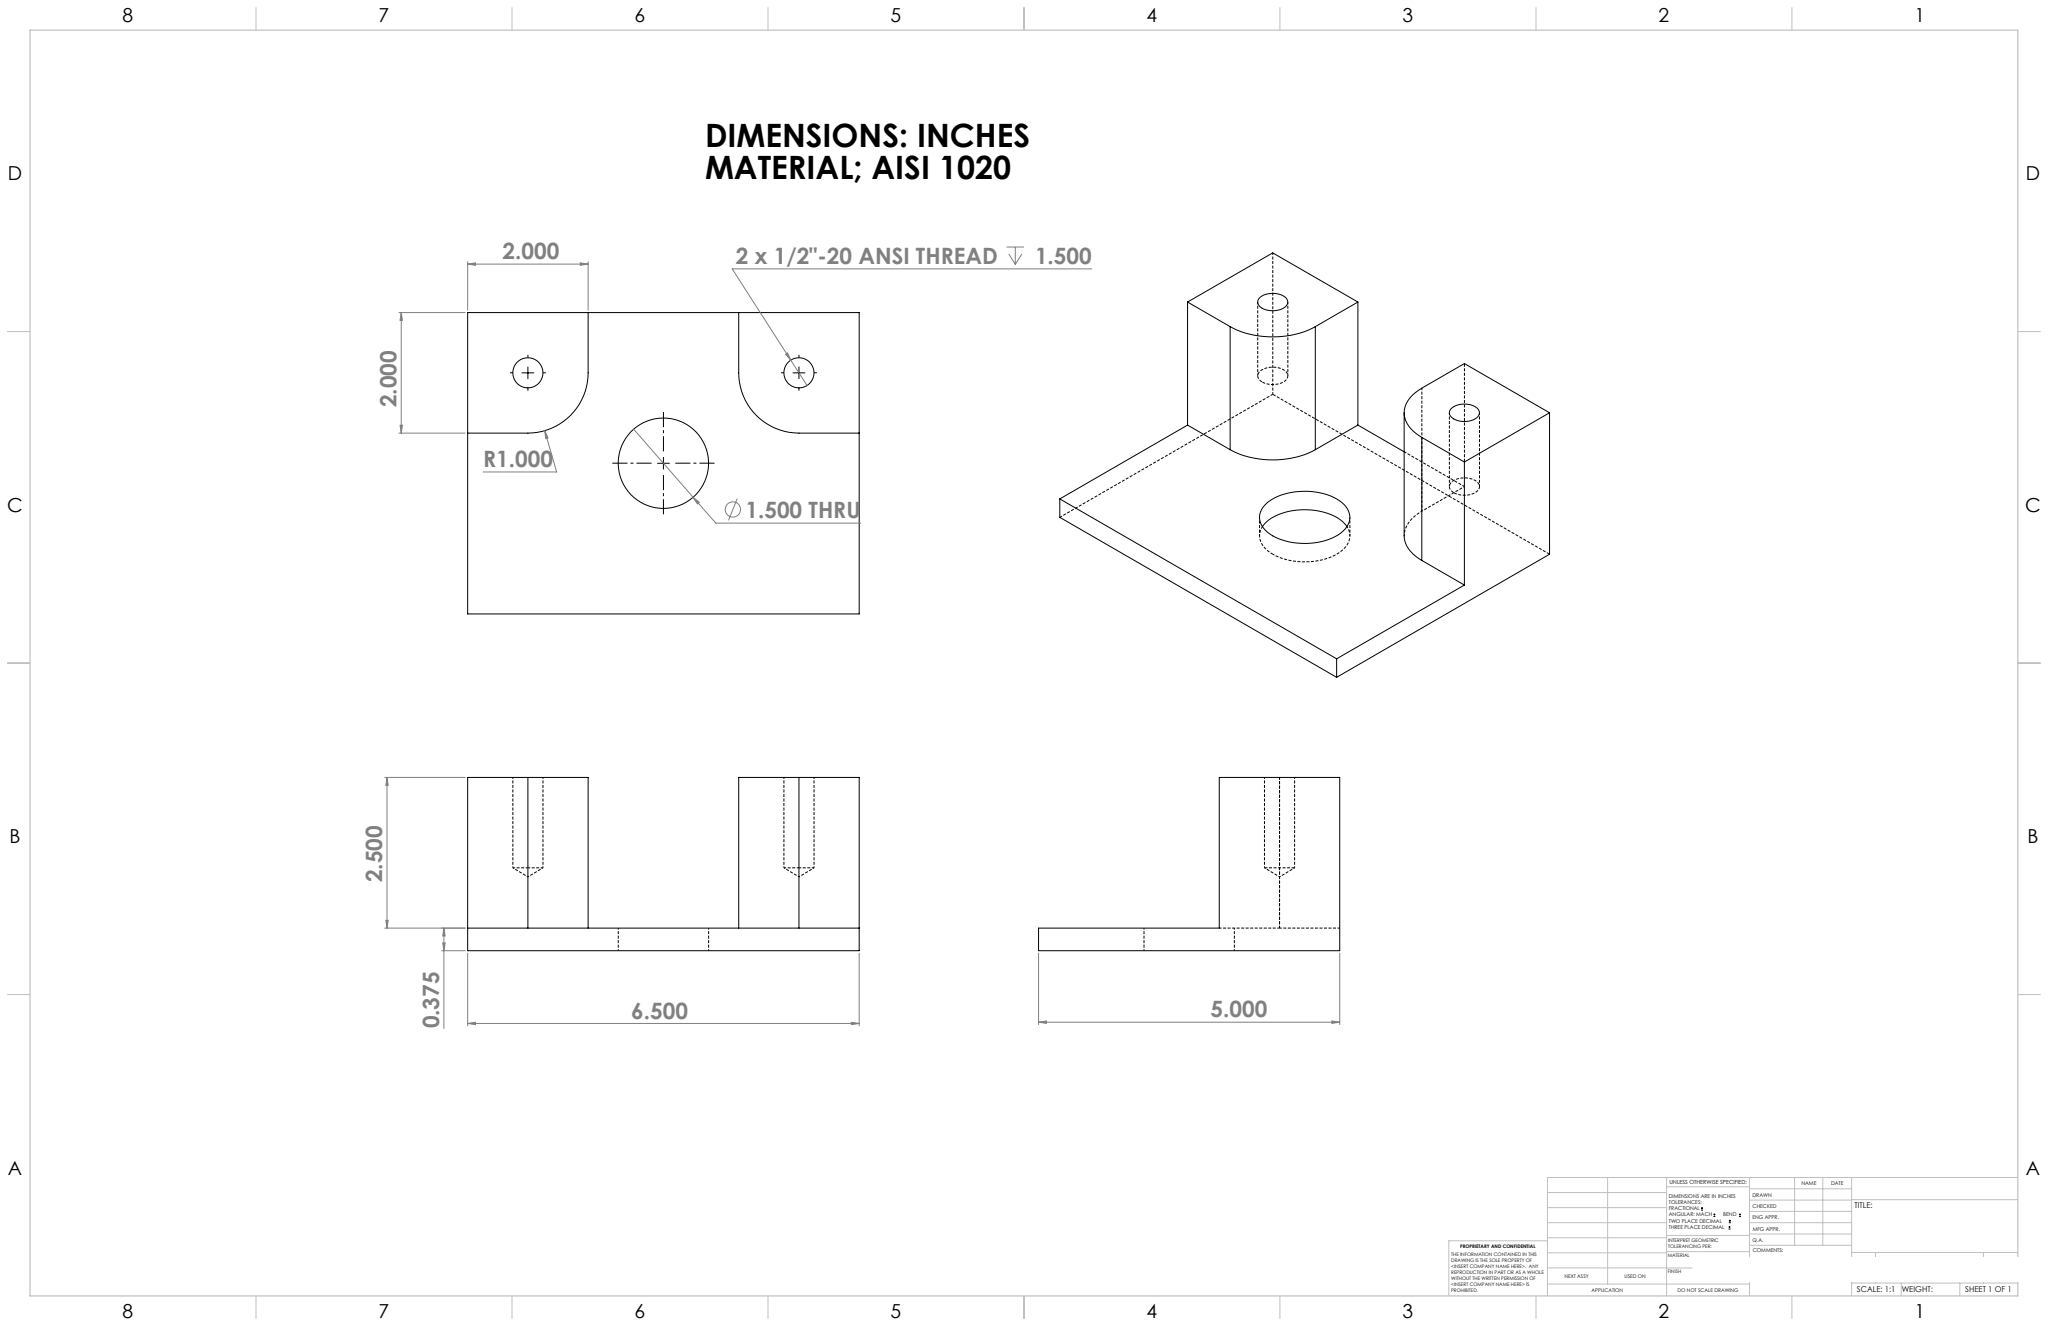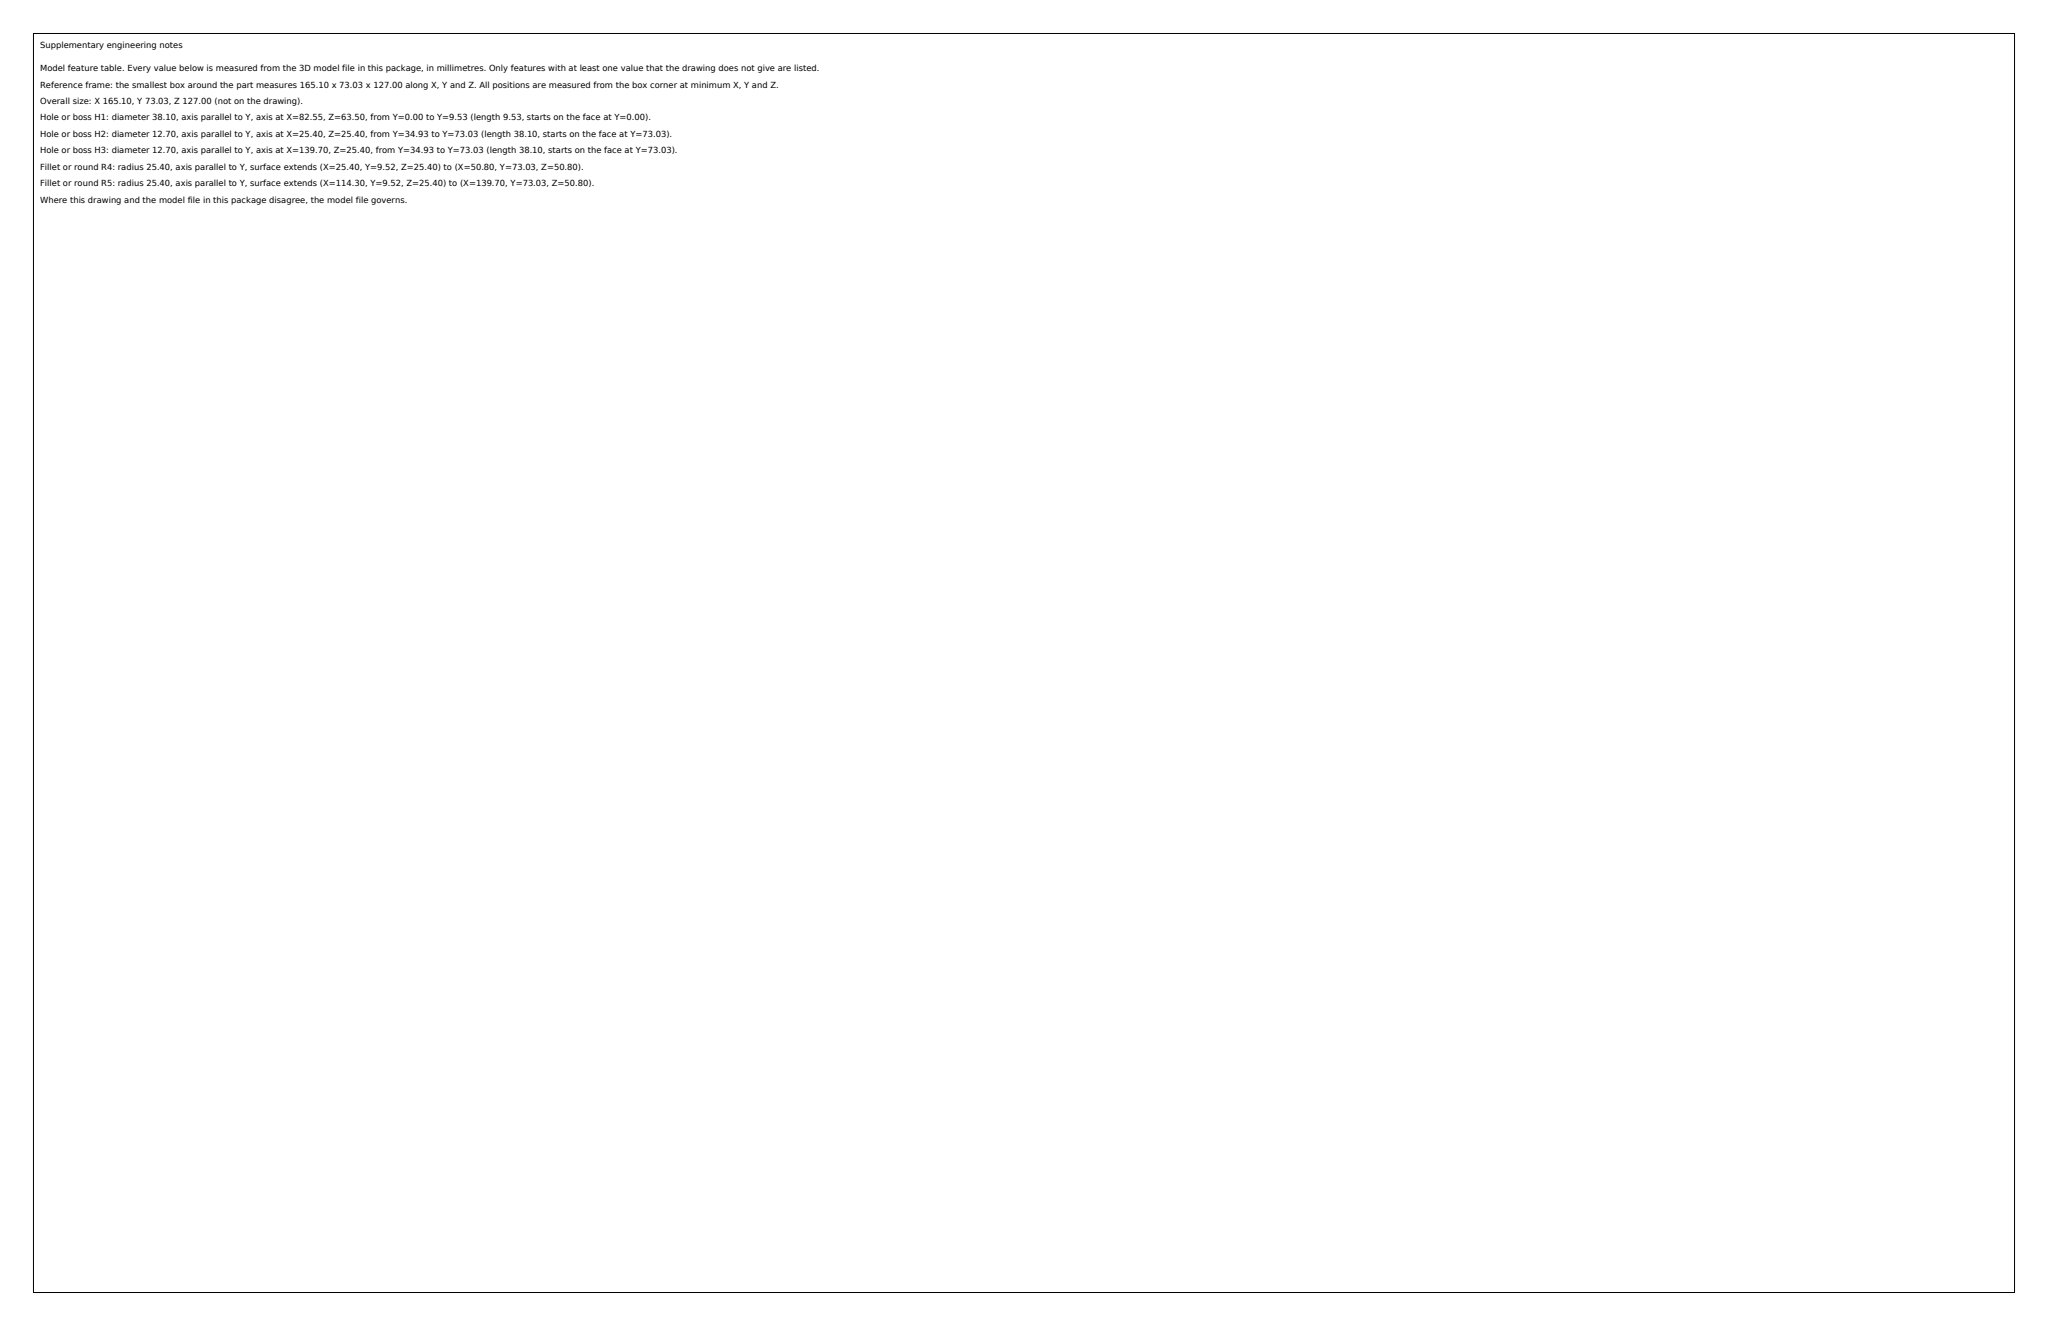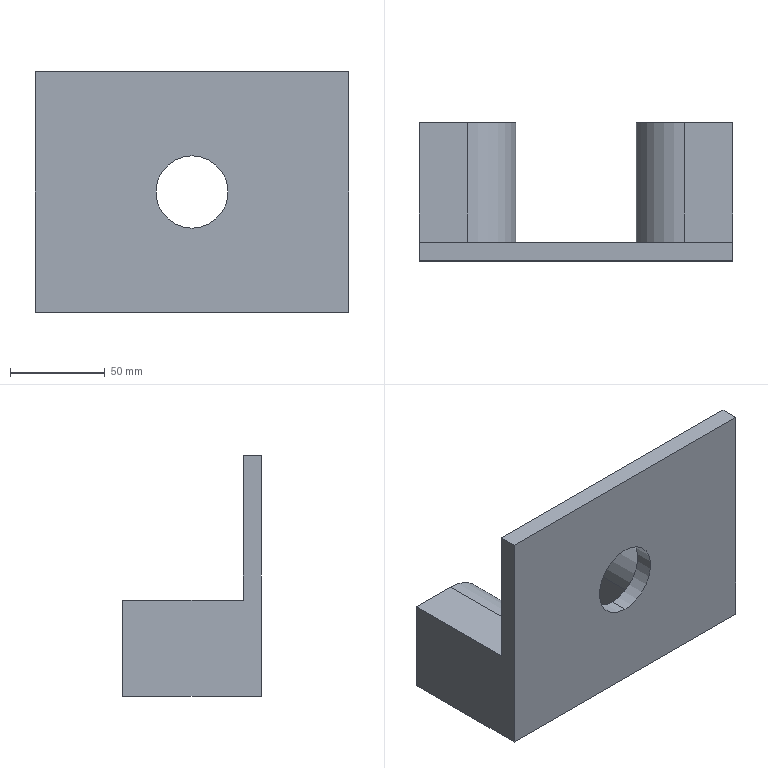Part | SolidWorks | mm | material AISI 1020 | 1 solid | 24 faces | box 165.1 x 73.03 x 127 mm | volume 489041 mm3 | plane 12 | cylinder 8 | cone 4 | commonest cylinder face diameters 12.7 x4 38.1 x2 50.8 x2
Drawing notes:
2 x 1/2-20 TAP CL: 1.000 FROM REAR & END EDGES, 4.500 APART | from the solid: Ø12.7 y-axis holes at (x,z)=(25.4,25.4) & (139.7,25.4); bbox 165.1 x 127.0; 139.7-25.4=114.3 (4.500 in), 25.4=1.000 in
build123d program:
from build123d import *

# Parameters (mm, degrees)
SKETCH1_W                      = 165.1
SKETCH1_H                      = 127
SKETCH1_R                      = 19.05
BOSS_EXTRUDE1_DEPTH            = 9.525
BOSS_EXTRUDE2_DEPTH            = 63.5
F_1_2_0_5_DIAMETER_HOLE1_D     = 12.7
F_1_2_0_5_DIAMETER_HOLE1_DEPTH = 38.1
F_1_2_0_5_DIAMETER_HOLE1_TIP   = 3.815


with BuildPart() as part:
    # Sketch1 → Boss-Extrude1 (new body)
    with BuildSketch(Plane(origin=(0, 0, 0), x_dir=(1, 0, 0), z_dir=(0, 1, 0))):
        Rectangle(SKETCH1_W, SKETCH1_H)
        with Locations(Location((0, 0, 0), (0, 0, 90))):
            Circle(SKETCH1_R, mode=Mode.SUBTRACT)
    extrude(amount=BOSS_EXTRUDE1_DEPTH)

    # Sketch2 → Boss-Extrude2 (add)
    with BuildSketch(Plane(origin=(0, 9.525, 0), x_dir=(1, 0, 0), z_dir=(0, 1, 0))):
        with BuildLine():
            Line((-82.55, 63.5), (-31.75, 63.5))
            Line((-31.75, 63.5), (-31.75, 38.1))
            ThreePointArc((-31.75, 38.1), (-39.189, 20.139), (-57.15, 12.7))
            Line((-57.15, 12.7), (-82.55, 12.7))
            Line((-82.55, 12.7), (-82.55, 63.5))
        make_face()
        with BuildLine():
            Line((31.75, 63.5), (31.75, 38.1))
            ThreePointArc((31.75, 38.1), (39.189, 20.139), (57.15, 12.7))
            Line((57.15, 12.7), (82.55, 12.7))
            Line((82.55, 12.7), (82.55, 63.5))
            Line((82.55, 63.5), (31.75, 63.5))
        make_face()
    extrude(amount=BOSS_EXTRUDE2_DEPTH)

    # 1_2 _0.5_ Diameter Hole1
    with Locations(Plane(origin=(0, 73.025, 0), x_dir=(1, 0, 0), z_dir=(0, 1, 0))):
        with Locations((-57.15, 38.1), (57.15, 38.1)):
            Hole(F_1_2_0_5_DIAMETER_HOLE1_D / 2, depth=F_1_2_0_5_DIAMETER_HOLE1_DEPTH)
            with Locations((0, 0, -(F_1_2_0_5_DIAMETER_HOLE1_DEPTH + F_1_2_0_5_DIAMETER_HOLE1_TIP / 2))):  # 118° drill point
                Cone(0, F_1_2_0_5_DIAMETER_HOLE1_D / 2, F_1_2_0_5_DIAMETER_HOLE1_TIP, mode=Mode.SUBTRACT)


solid = part.part
STEP:
#1=CARTESIAN_POINT('',(-2.25,1.375,-1.75));
#2=VERTEX_POINT('',#1);
#3=CARTESIAN_POINT('',(-2.25,1.375,-1.25));
#4=VERTEX_POINT('',#3);
#5=CARTESIAN_POINT('',(-2.25,1.375,-1.5));
#6=DIRECTION('',(0.,1.,0.));
#7=DIRECTION('',(0.,0.,1.));
#8=AXIS2_PLACEMENT_3D('',#5,#6,#7);
#9=CIRCLE('',#8,0.25);
#10=EDGE_CURVE('',#2,#4,#9,.T.);
#11=ORIENTED_EDGE('',*,*,#10,.F.);
#12=CARTESIAN_POINT('',(-2.25,2.875,-1.75));
#13=VERTEX_POINT('',#12);
#14=CARTESIAN_POINT('',(-2.25,2.875,-1.75));
#15=DIRECTION('',(0.,1.,0.));
#16=VECTOR('',#15,39.37);
#17=LINE('',#14,#16);
#18=EDGE_CURVE('',#2,#13,#17,.T.);
#19=ORIENTED_EDGE('',*,*,#18,.T.);
#20=CARTESIAN_POINT('',(-2.25,2.875,-1.25));
#21=VERTEX_POINT('',#20);
#22=CARTESIAN_POINT('',(-2.25,2.875,-1.5));
#23=DIRECTION('',(0.,1.,0.));
#24=DIRECTION('',(0.,0.,1.));
#25=AXIS2_PLACEMENT_3D('',#22,#23,#24);
#26=CIRCLE('',#25,0.25);
#27=EDGE_CURVE('',#13,#21,#26,.T.);
#28=ORIENTED_EDGE('',*,*,#27,.T.);
#29=CARTESIAN_POINT('',(-2.25,2.875,-1.25));
#30=DIRECTION('',(0.,1.,0.));
#31=VECTOR('',#30,39.37);
#32=LINE('',#29,#31);
#33=EDGE_CURVE('',#4,#21,#32,.T.);
#34=ORIENTED_EDGE('',*,*,#33,.F.);
#35=EDGE_LOOP('',(#11,#19,#28,#34));
#36=FACE_OUTER_BOUND('',#35,.T.);
#37=CARTESIAN_POINT('',(-2.25,2.875,-1.5));
#38=DIRECTION('',(0.,1.,0.));
#39=DIRECTION('',(0.,0.,1.));
#40=AXIS2_PLACEMENT_3D('',#37,#38,#39);
#41=CYLINDRICAL_SURFACE('',#40,0.25);
#42=ADVANCED_FACE('',(#36),#41,.F.);
#43=CARTESIAN_POINT('',(-2.25,1.225,-1.5));
#44=VERTEX_POINT('',#43);
#45=CARTESIAN_POINT('',(-2.25,1.375,-1.25));
#46=DIRECTION('',(0.,0.515,0.8572));
#47=VECTOR('',#46,39.37);
#48=LINE('',#45,#47);
#49=EDGE_CURVE('',#44,#4,#48,.T.);
#50=ORIENTED_EDGE('',*,*,#49,.F.);
#51=CARTESIAN_POINT('',(-2.25,1.375,-1.75));
#52=DIRECTION('',(0.,0.515,-0.8572));
#53=VECTOR('',#52,39.37);
#54=LINE('',#51,#53);
#55=EDGE_CURVE('',#44,#2,#54,.T.);
#56=ORIENTED_EDGE('',*,*,#55,.T.);
#57=ORIENTED_EDGE('',*,*,#10,.T.);
#58=EDGE_LOOP('',(#50,#56,#57));
#59=FACE_OUTER_BOUND('',#58,.T.);
#60=CARTESIAN_POINT('',(-2.25,1.375,-1.5));
#61=DIRECTION('',(0.,1.,0.));
#62=DIRECTION('',(0.,0.,1.));
#63=AXIS2_PLACEMENT_3D('',#60,#61,#62);
#64=CONICAL_SURFACE('',#63,0.25,1.03);
#65=ADVANCED_FACE('',(#59),#64,.F.);
#66=CARTESIAN_POINT('',(2.25,1.375,-1.75));
#67=VERTEX_POINT('',#66);
#68=CARTESIAN_POINT('',(2.25,1.375,-1.25));
#69=VERTEX_POINT('',#68);
#70=CARTESIAN_POINT('',(2.25,1.375,-1.5));
#71=DIRECTION('',(0.,1.,0.));
#72=DIRECTION('',(0.,0.,1.));
#73=AXIS2_PLACEMENT_3D('',#70,#71,#72);
#74=CIRCLE('',#73,0.25);
#75=EDGE_CURVE('',#67,#69,#74,.T.);
#76=ORIENTED_EDGE('',*,*,#75,.F.);
#77=CARTESIAN_POINT('',(2.25,2.875,-1.75));
#78=VERTEX_POINT('',#77);
#79=CARTESIAN_POINT('',(2.25,2.875,-1.75));
#80=DIRECTION('',(0.,1.,0.));
#81=VECTOR('',#80,39.37);
#82=LINE('',#79,#81);
#83=EDGE_CURVE('',#67,#78,#82,.T.);
#84=ORIENTED_EDGE('',*,*,#83,.T.);
#85=CARTESIAN_POINT('',(2.25,2.875,-1.25));
#86=VERTEX_POINT('',#85);
#87=CARTESIAN_POINT('',(2.25,2.875,-1.5));
#88=DIRECTION('',(0.,1.,0.));
#89=DIRECTION('',(0.,0.,1.));
#90=AXIS2_PLACEMENT_3D('',#87,#88,#89);
#91=CIRCLE('',#90,0.25);
#92=EDGE_CURVE('',#78,#86,#91,.T.);
#93=ORIENTED_EDGE('',*,*,#92,.T.);
#94=CARTESIAN_POINT('',(2.25,2.875,-1.25));
#95=DIRECTION('',(0.,1.,0.));
#96=VECTOR('',#95,39.37);
#97=LINE('',#94,#96);
#98=EDGE_CURVE('',#69,#86,#97,.T.);
#99=ORIENTED_EDGE('',*,*,#98,.F.);
#100=EDGE_LOOP('',(#76,#84,#93,#99));
#101=FACE_OUTER_BOUND('',#100,.T.);
#102=CARTESIAN_POINT('',(2.25,2.875,-1.5));
#103=DIRECTION('',(0.,1.,0.));
#104=DIRECTION('',(0.,0.,1.));
#105=AXIS2_PLACEMENT_3D('',#102,#103,#104);
#106=CYLINDRICAL_SURFACE('',#105,0.25);
#107=ADVANCED_FACE('',(#101),#106,.F.);
#108=CARTESIAN_POINT('',(2.25,1.225,-1.5));
#109=VERTEX_POINT('',#108);
#110=CARTESIAN_POINT('',(2.25,1.375,-1.25));
#111=DIRECTION('',(0.,0.515,0.8572));
#112=VECTOR('',#111,39.37);
#113=LINE('',#110,#112);
#114=EDGE_CURVE('',#109,#69,#113,.T.);
#115=ORIENTED_EDGE('',*,*,#114,.F.);
#116=CARTESIAN_POINT('',(2.25,1.375,-1.75));
#117=DIRECTION('',(0.,0.515,-0.8572));
#118=VECTOR('',#117,39.37);
#119=LINE('',#116,#118);
#120=EDGE_CURVE('',#109,#67,#119,.T.);
#121=ORIENTED_EDGE('',*,*,#120,.T.);
#122=ORIENTED_EDGE('',*,*,#75,.T.);
#123=EDGE_LOOP('',(#115,#121,#122));
#124=FACE_OUTER_BOUND('',#123,.T.);
#125=CARTESIAN_POINT('',(2.25,1.375,-1.5));
#126=DIRECTION('',(0.,1.,0.));
#127=DIRECTION('',(0.,0.,1.));
#128=AXIS2_PLACEMENT_3D('',#125,#126,#127);
#129=CONICAL_SURFACE('',#128,0.25,1.03);
#130=ADVANCED_FACE('',(#124),#129,.F.);
#131=CARTESIAN_POINT('',(0.,0.375,-0.75));
#132=VERTEX_POINT('',#131);
#133=CARTESIAN_POINT('',(0.,0.375,0.75));
#134=VERTEX_POINT('',#133);
#135=CARTESIAN_POINT('',(0.,0.375,-0.));
#136=DIRECTION('',(0.,1.,0.));
#137=DIRECTION('',(0.,0.,1.));
#138=AXIS2_PLACEMENT_3D('',#135,#136,#137);
#139=CIRCLE('',#138,0.75);
#140=EDGE_CURVE('',#132,#134,#139,.T.);
#141=ORIENTED_EDGE('',*,*,#140,.T.);
#142=CARTESIAN_POINT('',(0.,0.,0.75));
#143=VERTEX_POINT('',#142);
#144=CARTESIAN_POINT('',(0.,0.375,0.75));
#145=DIRECTION('',(0.,-1.,0.));
#146=VECTOR('',#145,39.37);
#147=LINE('',#144,#146);
#148=EDGE_CURVE('',#134,#143,#147,.T.);
#149=ORIENTED_EDGE('',*,*,#148,.T.);
#150=CARTESIAN_POINT('',(0.,0.,-0.75));
#151=VERTEX_POINT('',#150);
#152=CARTESIAN_POINT('',(0.,0.,-0.));
#153=DIRECTION('',(0.,1.,0.));
#154=DIRECTION('',(0.,0.,1.));
#155=AXIS2_PLACEMENT_3D('',#152,#153,#154);
#156=CIRCLE('',#155,0.75);
#157=EDGE_CURVE('',#151,#143,#156,.T.);
#158=ORIENTED_EDGE('',*,*,#157,.F.);
#159=CARTESIAN_POINT('',(0.,0.375,-0.75));
#160=DIRECTION('',(0.,-1.,0.));
#161=VECTOR('',#160,39.37);
#162=LINE('',#159,#161);
#163=EDGE_CURVE('',#132,#151,#162,.T.);
#164=ORIENTED_EDGE('',*,*,#163,.F.);
#165=EDGE_LOOP('',(#141,#149,#158,#164));
#166=FACE_OUTER_BOUND('',#165,.T.);
#167=CARTESIAN_POINT('',(0.,0.375,-0.));
#168=DIRECTION('',(0.,-1.,0.));
#169=DIRECTION('',(0.,0.,-1.));
#170=AXIS2_PLACEMENT_3D('',#167,#168,#169);
#171=CYLINDRICAL_SURFACE('',#170,0.75);
#172=ADVANCED_FACE('',(#166),#171,.F.);
#173=ORIENTED_EDGE('',*,*,#140,.F.);
#174=CARTESIAN_POINT('',(0.,0.375,-0.));
#175=DIRECTION('',(0.,1.,0.));
#176=DIRECTION('',(0.,0.,1.));
#177=AXIS2_PLACEMENT_3D('',#174,#175,#176);
#178=CIRCLE('',#177,0.75);
#179=EDGE_CURVE('',#134,#132,#178,.T.);
#180=ORIENTED_EDGE('',*,*,#179,.F.);
#181=EDGE_LOOP('',(#173,#180));
#182=FACE_BOUND('',#181,.T.);
#183=CARTESIAN_POINT('',(-1.25,0.375,-1.5));
#184=VERTEX_POINT('',#183);
#185=CARTESIAN_POINT('',(-1.25,0.375,-2.5));
#186=VERTEX_POINT('',#185);
#187=CARTESIAN_POINT('',(-1.25,0.375,-2.5));
#188=DIRECTION('',(0.,0.,-1.));
#189=VECTOR('',#188,39.37);
#190=LINE('',#187,#189);
#191=EDGE_CURVE('',#184,#186,#190,.T.);
#192=ORIENTED_EDGE('',*,*,#191,.F.);
#193=CARTESIAN_POINT('',(-2.25,0.375,-0.5));
#194=VERTEX_POINT('',#193);
#195=CARTESIAN_POINT('',(-2.25,0.375,-1.5));
#196=DIRECTION('',(0.,1.,0.));
#197=DIRECTION('',(0.,0.,1.));
#198=AXIS2_PLACEMENT_3D('',#195,#196,#197);
#199=CIRCLE('',#198,1.);
#200=EDGE_CURVE('',#194,#184,#199,.T.);
#201=ORIENTED_EDGE('',*,*,#200,.F.);
#202=CARTESIAN_POINT('',(-3.25,0.375,-0.5));
#203=VERTEX_POINT('',#202);
#204=CARTESIAN_POINT('',(-3.25,0.375,-0.5));
#205=DIRECTION('',(1.,0.,0.));
#206=VECTOR('',#205,39.37);
#207=LINE('',#204,#206);
#208=EDGE_CURVE('',#203,#194,#207,.T.);
#209=ORIENTED_EDGE('',*,*,#208,.F.);
#210=CARTESIAN_POINT('',(-3.25,0.375,2.5));
#211=VERTEX_POINT('',#210);
#212=CARTESIAN_POINT('',(-3.25,0.375,2.5));
#213=DIRECTION('',(0.,0.,1.));
#214=VECTOR('',#213,39.37);
#215=LINE('',#212,#214);
#216=EDGE_CURVE('',#203,#211,#215,.T.);
#217=ORIENTED_EDGE('',*,*,#216,.T.);
#218=CARTESIAN_POINT('',(3.25,0.375,2.5));
#219=VERTEX_POINT('',#218);
#220=CARTESIAN_POINT('',(-3.25,0.375,2.5));
#221=DIRECTION('',(1.,0.,0.));
#222=VECTOR('',#221,39.37);
#223=LINE('',#220,#222);
#224=EDGE_CURVE('',#211,#219,#223,.T.);
#225=ORIENTED_EDGE('',*,*,#224,.T.);
#226=CARTESIAN_POINT('',(3.25,0.375,-0.5));
#227=VERTEX_POINT('',#226);
#228=CARTESIAN_POINT('',(3.25,0.375,2.5));
#229=DIRECTION('',(0.,0.,-1.));
#230=VECTOR('',#229,39.37);
#231=LINE('',#228,#230);
#232=EDGE_CURVE('',#219,#227,#231,.T.);
#233=ORIENTED_EDGE('',*,*,#232,.T.);
#234=CARTESIAN_POINT('',(2.25,0.375,-0.5));
#235=VERTEX_POINT('',#234);
#236=CARTESIAN_POINT('',(3.25,0.375,-0.5));
#237=DIRECTION('',(1.,0.,0.));
#238=VECTOR('',#237,39.37);
#239=LINE('',#236,#238);
#240=EDGE_CURVE('',#235,#227,#239,.T.);
#241=ORIENTED_EDGE('',*,*,#240,.F.);
#242=CARTESIAN_POINT('',(1.25,0.375,-1.5));
#243=VERTEX_POINT('',#242);
#244=CARTESIAN_POINT('',(2.25,0.375,-1.5));
#245=DIRECTION('',(0.,1.,0.));
#246=DIRECTION('',(0.,0.,-1.));
#247=AXIS2_PLACEMENT_3D('',#244,#245,#246);
#248=CIRCLE('',#247,1.);
#249=EDGE_CURVE('',#243,#235,#248,.T.);
#250=ORIENTED_EDGE('',*,*,#249,.F.);
#251=CARTESIAN_POINT('',(1.25,0.375,-2.5));
#252=VERTEX_POINT('',#251);
#253=CARTESIAN_POINT('',(1.25,0.375,-2.5));
#254=DIRECTION('',(0.,0.,1.));
#255=VECTOR('',#254,39.37);
#256=LINE('',#253,#255);
#257=EDGE_CURVE('',#252,#243,#256,.T.);
#258=ORIENTED_EDGE('',*,*,#257,.F.);
#259=CARTESIAN_POINT('',(-3.25,0.375,-2.5));
#260=DIRECTION('',(-1.,0.,0.));
#261=VECTOR('',#260,39.37);
#262=LINE('',#259,#261);
#263=EDGE_CURVE('',#252,#186,#262,.T.);
#264=ORIENTED_EDGE('',*,*,#263,.T.);
#265=EDGE_LOOP('',(#192,#201,#209,#217,#225,#233,#241,#250,#258,#264));
#266=FACE_OUTER_BOUND('',#265,.T.);
#267=CARTESIAN_POINT('',(0.,0.375,0.));
#268=DIRECTION('',(0.,-1.,0.));
#269=DIRECTION('',(0.,0.,-1.));
#270=AXIS2_PLACEMENT_3D('',#267,#268,#269);
#271=PLANE('',#270);
#272=ADVANCED_FACE('',(#182,#266),#271,.F.);
#273=CARTESIAN_POINT('',(3.25,0.,2.5));
#274=VERTEX_POINT('',#273);
#275=CARTESIAN_POINT('',(3.25,0.,-2.5));
#276=VERTEX_POINT('',#275);
#277=CARTESIAN_POINT('',(3.25,0.,2.5));
#278=DIRECTION('',(0.,0.,-1.));
#279=VECTOR('',#278,39.37);
#280=LINE('',#277,#279);
#281=EDGE_CURVE('',#274,#276,#280,.T.);
#282=ORIENTED_EDGE('',*,*,#281,.F.);
#283=CARTESIAN_POINT('',(-3.25,0.,2.5));
#284=VERTEX_POINT('',#283);
#285=CARTESIAN_POINT('',(-3.25,0.,2.5));
#286=DIRECTION('',(1.,0.,0.));
#287=VECTOR('',#286,39.37);
#288=LINE('',#285,#287);
#289=EDGE_CURVE('',#284,#274,#288,.T.);
#290=ORIENTED_EDGE('',*,*,#289,.F.);
#291=CARTESIAN_POINT('',(-3.25,0.,-2.5));
#292=VERTEX_POINT('',#291);
#293=CARTESIAN_POINT('',(-3.25,0.,2.5));
#294=DIRECTION('',(0.,0.,1.));
#295=VECTOR('',#294,39.37);
#296=LINE('',#293,#295);
#297=EDGE_CURVE('',#292,#284,#296,.T.);
#298=ORIENTED_EDGE('',*,*,#297,.F.);
#299=CARTESIAN_POINT('',(-3.25,0.,-2.5));
#300=DIRECTION('',(-1.,0.,0.));
#301=VECTOR('',#300,39.37);
#302=LINE('',#299,#301);
#303=EDGE_CURVE('',#276,#292,#302,.T.);
#304=ORIENTED_EDGE('',*,*,#303,.F.);
#305=EDGE_LOOP('',(#282,#290,#298,#304));
#306=FACE_OUTER_BOUND('',#305,.T.);
#307=ORIENTED_EDGE('',*,*,#157,.T.);
#308=CARTESIAN_POINT('',(0.,0.,-0.));
#309=DIRECTION('',(0.,1.,0.));
#310=DIRECTION('',(0.,0.,1.));
#311=AXIS2_PLACEMENT_3D('',#308,#309,#310);
#312=CIRCLE('',#311,0.75);
#313=EDGE_CURVE('',#143,#151,#312,.T.);
#314=ORIENTED_EDGE('',*,*,#313,.T.);
#315=EDGE_LOOP('',(#307,#314));
#316=FACE_BOUND('',#315,.T.);
#317=CARTESIAN_POINT('',(0.,0.,0.));
#318=DIRECTION('',(0.,-1.,0.));
#319=DIRECTION('',(0.,0.,-1.));
#320=AXIS2_PLACEMENT_3D('',#317,#318,#319);
#321=PLANE('',#320);
#322=ADVANCED_FACE('',(#306,#316),#321,.T.);
#323=ORIENTED_EDGE('',*,*,#281,.T.);
#324=CARTESIAN_POINT('',(3.25,2.875,-2.5));
#325=VERTEX_POINT('',#324);
#326=CARTESIAN_POINT('',(3.25,0.375,-2.5));
#327=DIRECTION('',(0.,-1.,0.));
#328=VECTOR('',#327,39.37);
#329=LINE('',#326,#328);
#330=EDGE_CURVE('',#325,#276,#329,.T.);
#331=ORIENTED_EDGE('',*,*,#330,.F.);
#332=CARTESIAN_POINT('',(3.25,2.875,-0.5));
#333=VERTEX_POINT('',#332);
#334=CARTESIAN_POINT('',(3.25,2.875,-2.5));
#335=DIRECTION('',(0.,0.,-1.));
#336=VECTOR('',#335,39.37);
#337=LINE('',#334,#336);
#338=EDGE_CURVE('',#333,#325,#337,.T.);
#339=ORIENTED_EDGE('',*,*,#338,.F.);
#340=CARTESIAN_POINT('',(3.25,2.875,-0.5));
#341=DIRECTION('',(0.,-1.,0.));
#342=VECTOR('',#341,39.37);
#343=LINE('',#340,#342);
#344=EDGE_CURVE('',#333,#227,#343,.T.);
#345=ORIENTED_EDGE('',*,*,#344,.T.);
#346=ORIENTED_EDGE('',*,*,#232,.F.);
#347=CARTESIAN_POINT('',(3.25,0.375,2.5));
#348=DIRECTION('',(0.,-1.,0.));
#349=VECTOR('',#348,39.37);
#350=LINE('',#347,#349);
#351=EDGE_CURVE('',#219,#274,#350,.T.);
#352=ORIENTED_EDGE('',*,*,#351,.T.);
#353=EDGE_LOOP('',(#323,#331,#339,#345,#346,#352));
#354=FACE_OUTER_BOUND('',#353,.T.);
#355=CARTESIAN_POINT('',(3.25,0.375,2.5));
#356=DIRECTION('',(-1.,0.,0.));
#357=DIRECTION('',(0.,0.,1.));
#358=AXIS2_PLACEMENT_3D('',#355,#356,#357);
#359=PLANE('',#358);
#360=ADVANCED_FACE('',(#354),#359,.F.);
#361=ORIENTED_EDGE('',*,*,#303,.T.);
#362=CARTESIAN_POINT('',(-3.25,2.875,-2.5));
#363=VERTEX_POINT('',#362);
#364=CARTESIAN_POINT('',(-3.25,0.375,-2.5));
#365=DIRECTION('',(0.,-1.,0.));
#366=VECTOR('',#365,39.37);
#367=LINE('',#364,#366);
#368=EDGE_CURVE('',#363,#292,#367,.T.);
#369=ORIENTED_EDGE('',*,*,#368,.F.);
#370=CARTESIAN_POINT('',(-1.25,2.875,-2.5));
#371=VERTEX_POINT('',#370);
#372=CARTESIAN_POINT('',(-3.25,2.875,-2.5));
#373=DIRECTION('',(-1.,0.,0.));
#374=VECTOR('',#373,39.37);
#375=LINE('',#372,#374);
#376=EDGE_CURVE('',#371,#363,#375,.T.);
#377=ORIENTED_EDGE('',*,*,#376,.F.);
#378=CARTESIAN_POINT('',(-1.25,2.875,-2.5));
#379=DIRECTION('',(0.,-1.,0.));
#380=VECTOR('',#379,39.37);
#381=LINE('',#378,#380);
#382=EDGE_CURVE('',#371,#186,#381,.T.);
#383=ORIENTED_EDGE('',*,*,#382,.T.);
#384=ORIENTED_EDGE('',*,*,#263,.F.);
#385=CARTESIAN_POINT('',(1.25,2.875,-2.5));
#386=VERTEX_POINT('',#385);
#387=CARTESIAN_POINT('',(1.25,2.875,-2.5));
#388=DIRECTION('',(0.,-1.,0.));
#389=VECTOR('',#388,39.37);
#390=LINE('',#387,#389);
#391=EDGE_CURVE('',#386,#252,#390,.T.);
#392=ORIENTED_EDGE('',*,*,#391,.F.);
#393=CARTESIAN_POINT('',(3.25,2.875,-2.5));
#394=DIRECTION('',(-1.,0.,0.));
#395=VECTOR('',#394,39.37);
#396=LINE('',#393,#395);
#397=EDGE_CURVE('',#325,#386,#396,.T.);
#398=ORIENTED_EDGE('',*,*,#397,.F.);
#399=ORIENTED_EDGE('',*,*,#330,.T.);
#400=EDGE_LOOP('',(#361,#369,#377,#383,#384,#392,#398,#399));
#401=FACE_OUTER_BOUND('',#400,.T.);
#402=CARTESIAN_POINT('',(-3.25,0.375,-2.5));
#403=DIRECTION('',(0.,0.,1.));
#404=DIRECTION('',(1.,0.,0.));
#405=AXIS2_PLACEMENT_3D('',#402,#403,#404);
#406=PLANE('',#405);
#407=ADVANCED_FACE('',(#401),#406,.F.);
#408=ORIENTED_EDGE('',*,*,#297,.T.);
#409=CARTESIAN_POINT('',(-3.25,0.375,2.5));
#410=DIRECTION('',(0.,-1.,0.));
#411=VECTOR('',#410,39.37);
#412=LINE('',#409,#411);
#413=EDGE_CURVE('',#211,#284,#412,.T.);
#414=ORIENTED_EDGE('',*,*,#413,.F.);
#415=ORIENTED_EDGE('',*,*,#216,.F.);
#416=CARTESIAN_POINT('',(-3.25,2.875,-0.5));
#417=VERTEX_POINT('',#416);
#418=CARTESIAN_POINT('',(-3.25,2.875,-0.5));
#419=DIRECTION('',(0.,-1.,0.));
#420=VECTOR('',#419,39.37);
#421=LINE('',#418,#420);
#422=EDGE_CURVE('',#417,#203,#421,.T.);
#423=ORIENTED_EDGE('',*,*,#422,.F.);
#424=CARTESIAN_POINT('',(-3.25,2.875,-2.5));
#425=DIRECTION('',(0.,0.,1.));
#426=VECTOR('',#425,39.37);
#427=LINE('',#424,#426);
#428=EDGE_CURVE('',#363,#417,#427,.T.);
#429=ORIENTED_EDGE('',*,*,#428,.F.);
#430=ORIENTED_EDGE('',*,*,#368,.T.);
#431=EDGE_LOOP('',(#408,#414,#415,#423,#429,#430));
#432=FACE_OUTER_BOUND('',#431,.T.);
#433=CARTESIAN_POINT('',(-3.25,0.375,2.5));
#434=DIRECTION('',(1.,0.,0.));
#435=DIRECTION('',(0.,0.,-1.));
#436=AXIS2_PLACEMENT_3D('',#433,#434,#435);
#437=PLANE('',#436);
#438=ADVANCED_FACE('',(#432),#437,.F.);
#439=ORIENTED_EDGE('',*,*,#289,.T.);
#440=ORIENTED_EDGE('',*,*,#351,.F.);
#441=ORIENTED_EDGE('',*,*,#224,.F.);
#442=ORIENTED_EDGE('',*,*,#413,.T.);
#443=EDGE_LOOP('',(#439,#440,#441,#442));
#444=FACE_OUTER_BOUND('',#443,.T.);
#445=CARTESIAN_POINT('',(-3.25,0.375,2.5));
#446=DIRECTION('',(0.,0.,-1.));
#447=DIRECTION('',(-1.,0.,0.));
#448=AXIS2_PLACEMENT_3D('',#445,#446,#447);
#449=PLANE('',#448);
#450=ADVANCED_FACE('',(#444),#449,.F.);
#451=ORIENTED_EDGE('',*,*,#148,.F.);
#452=ORIENTED_EDGE('',*,*,#179,.T.);
#453=ORIENTED_EDGE('',*,*,#163,.T.);
#454=ORIENTED_EDGE('',*,*,#313,.F.);
#455=EDGE_LOOP('',(#451,#452,#453,#454));
#456=FACE_OUTER_BOUND('',#455,.T.);
#457=CARTESIAN_POINT('',(0.,0.375,-0.));
#458=DIRECTION('',(0.,-1.,0.));
#459=DIRECTION('',(0.,0.,-1.));
#460=AXIS2_PLACEMENT_3D('',#457,#458,#459);
#461=CYLINDRICAL_SURFACE('',#460,0.75);
#462=ADVANCED_FACE('',(#456),#461,.F.);
#463=ORIENTED_EDGE('',*,*,#249,.T.);
#464=CARTESIAN_POINT('',(2.25,2.875,-0.5));
#465=VERTEX_POINT('',#464);
#466=CARTESIAN_POINT('',(2.25,2.875,-0.5));
#467=DIRECTION('',(0.,-1.,0.));
#468=VECTOR('',#467,39.37);
#469=LINE('',#466,#468);
#470=EDGE_CURVE('',#465,#235,#469,.T.);
#471=ORIENTED_EDGE('',*,*,#470,.F.);
#472=CARTESIAN_POINT('',(1.25,2.875,-1.5));
#473=VERTEX_POINT('',#472);
#474=CARTESIAN_POINT('',(2.25,2.875,-1.5));
#475=DIRECTION('',(0.,1.,0.));
#476=DIRECTION('',(0.,0.,-1.));
#477=AXIS2_PLACEMENT_3D('',#474,#475,#476);
#478=CIRCLE('',#477,1.);
#479=EDGE_CURVE('',#473,#465,#478,.T.);
#480=ORIENTED_EDGE('',*,*,#479,.F.);
#481=CARTESIAN_POINT('',(1.25,2.875,-1.5));
#482=DIRECTION('',(0.,-1.,0.));
#483=VECTOR('',#482,39.37);
#484=LINE('',#481,#483);
#485=EDGE_CURVE('',#473,#243,#484,.T.);
#486=ORIENTED_EDGE('',*,*,#485,.T.);
#487=EDGE_LOOP('',(#463,#471,#480,#486));
#488=FACE_OUTER_BOUND('',#487,.T.);
#489=CARTESIAN_POINT('',(2.25,2.875,-1.5));
#490=DIRECTION('',(0.,-1.,0.));
#491=DIRECTION('',(0.,0.,-1.));
#492=AXIS2_PLACEMENT_3D('',#489,#490,#491);
#493=CYLINDRICAL_SURFACE('',#492,1.);
#494=ADVANCED_FACE('',(#488),#493,.T.);
#495=ORIENTED_EDGE('',*,*,#240,.T.);
#496=ORIENTED_EDGE('',*,*,#344,.F.);
#497=CARTESIAN_POINT('',(3.25,2.875,-0.5));
#498=DIRECTION('',(1.,0.,0.));
#499=VECTOR('',#498,39.37);
#500=LINE('',#497,#499);
#501=EDGE_CURVE('',#465,#333,#500,.T.);
#502=ORIENTED_EDGE('',*,*,#501,.F.);
#503=ORIENTED_EDGE('',*,*,#470,.T.);
#504=EDGE_LOOP('',(#495,#496,#502,#503));
#505=FACE_OUTER_BOUND('',#504,.T.);
#506=CARTESIAN_POINT('',(3.25,2.875,-0.5));
#507=DIRECTION('',(0.,0.,-1.));
#508=DIRECTION('',(-1.,0.,0.));
#509=AXIS2_PLACEMENT_3D('',#506,#507,#508);
#510=PLANE('',#509);
#511=ADVANCED_FACE('',(#505),#510,.F.);
#512=ORIENTED_EDGE('',*,*,#257,.T.);
#513=ORIENTED_EDGE('',*,*,#485,.F.);
#514=CARTESIAN_POINT('',(1.25,2.875,-2.5));
#515=DIRECTION('',(0.,0.,1.));
#516=VECTOR('',#515,39.37);
#517=LINE('',#514,#516);
#518=EDGE_CURVE('',#386,#473,#517,.T.);
#519=ORIENTED_EDGE('',*,*,#518,.F.);
#520=ORIENTED_EDGE('',*,*,#391,.T.);
#521=EDGE_LOOP('',(#512,#513,#519,#520));
#522=FACE_OUTER_BOUND('',#521,.T.);
#523=CARTESIAN_POINT('',(1.25,2.875,-2.5));
#524=DIRECTION('',(1.,0.,0.));
#525=DIRECTION('',(0.,0.,-1.));
#526=AXIS2_PLACEMENT_3D('',#523,#524,#525);
#527=PLANE('',#526);
#528=ADVANCED_FACE('',(#522),#527,.F.);
#529=CARTESIAN_POINT('',(2.25,2.875,-1.5));
#530=DIRECTION('',(0.,1.,0.));
#531=DIRECTION('',(0.,0.,1.));
#532=AXIS2_PLACEMENT_3D('',#529,#530,#531);
#533=CIRCLE('',#532,0.25);
#534=EDGE_CURVE('',#86,#78,#533,.T.);
#535=ORIENTED_EDGE('',*,*,#534,.F.);
#536=ORIENTED_EDGE('',*,*,#92,.F.);
#537=EDGE_LOOP('',(#535,#536));
#538=FACE_BOUND('',#537,.T.);
#539=ORIENTED_EDGE('',*,*,#479,.T.);
#540=ORIENTED_EDGE('',*,*,#501,.T.);
#541=ORIENTED_EDGE('',*,*,#338,.T.);
#542=ORIENTED_EDGE('',*,*,#397,.T.);
#543=ORIENTED_EDGE('',*,*,#518,.T.);
#544=EDGE_LOOP('',(#539,#540,#541,#542,#543));
#545=FACE_OUTER_BOUND('',#544,.T.);
#546=CARTESIAN_POINT('',(2.25,2.875,-1.5));
#547=DIRECTION('',(0.,-1.,0.));
#548=DIRECTION('',(0.,0.,-1.));
#549=AXIS2_PLACEMENT_3D('',#546,#547,#548);
#550=PLANE('',#549);
#551=ADVANCED_FACE('',(#538,#545),#550,.F.);
#552=ORIENTED_EDGE('',*,*,#208,.T.);
#553=CARTESIAN_POINT('',(-2.25,2.875,-0.5));
#554=VERTEX_POINT('',#553);
#555=CARTESIAN_POINT('',(-2.25,2.875,-0.5));
#556=DIRECTION('',(0.,-1.,0.));
#557=VECTOR('',#556,39.37);
#558=LINE('',#555,#557);
#559=EDGE_CURVE('',#554,#194,#558,.T.);
#560=ORIENTED_EDGE('',*,*,#559,.F.);
#561=CARTESIAN_POINT('',(-3.25,2.875,-0.5));
#562=DIRECTION('',(1.,0.,0.));
#563=VECTOR('',#562,39.37);
#564=LINE('',#561,#563);
#565=EDGE_CURVE('',#417,#554,#564,.T.);
#566=ORIENTED_EDGE('',*,*,#565,.F.);
#567=ORIENTED_EDGE('',*,*,#422,.T.);
#568=EDGE_LOOP('',(#552,#560,#566,#567));
#569=FACE_OUTER_BOUND('',#568,.T.);
#570=CARTESIAN_POINT('',(-3.25,2.875,-0.5));
#571=DIRECTION('',(0.,0.,-1.));
#572=DIRECTION('',(-1.,0.,0.));
#573=AXIS2_PLACEMENT_3D('',#570,#571,#572);
#574=PLANE('',#573);
#575=ADVANCED_FACE('',(#569),#574,.F.);
#576=ORIENTED_EDGE('',*,*,#200,.T.);
#577=CARTESIAN_POINT('',(-1.25,2.875,-1.5));
#578=VERTEX_POINT('',#577);
#579=CARTESIAN_POINT('',(-1.25,2.875,-1.5));
#580=DIRECTION('',(0.,-1.,0.));
#581=VECTOR('',#580,39.37);
#582=LINE('',#579,#581);
#583=EDGE_CURVE('',#578,#184,#582,.T.);
#584=ORIENTED_EDGE('',*,*,#583,.F.);
#585=CARTESIAN_POINT('',(-2.25,2.875,-1.5));
#586=DIRECTION('',(0.,1.,0.));
#587=DIRECTION('',(0.,0.,1.));
#588=AXIS2_PLACEMENT_3D('',#585,#586,#587);
#589=CIRCLE('',#588,1.);
#590=EDGE_CURVE('',#554,#578,#589,.T.);
#591=ORIENTED_EDGE('',*,*,#590,.F.);
#592=ORIENTED_EDGE('',*,*,#559,.T.);
#593=EDGE_LOOP('',(#576,#584,#591,#592));
#594=FACE_OUTER_BOUND('',#593,.T.);
#595=CARTESIAN_POINT('',(-2.25,2.875,-1.5));
#596=DIRECTION('',(0.,-1.,0.));
#597=DIRECTION('',(0.,0.,-1.));
#598=AXIS2_PLACEMENT_3D('',#595,#596,#597);
#599=CYLINDRICAL_SURFACE('',#598,1.);
#600=ADVANCED_FACE('',(#594),#599,.T.);
#601=ORIENTED_EDGE('',*,*,#191,.T.);
#602=ORIENTED_EDGE('',*,*,#382,.F.);
#603=CARTESIAN_POINT('',(-1.25,2.875,-2.5));
#604=DIRECTION('',(0.,0.,-1.));
#605=VECTOR('',#604,39.37);
#606=LINE('',#603,#605);
#607=EDGE_CURVE('',#578,#371,#606,.T.);
#608=ORIENTED_EDGE('',*,*,#607,.F.);
#609=ORIENTED_EDGE('',*,*,#583,.T.);
#610=EDGE_LOOP('',(#601,#602,#608,#609));
#611=FACE_OUTER_BOUND('',#610,.T.);
#612=CARTESIAN_POINT('',(-1.25,2.875,-2.5));
#613=DIRECTION('',(-1.,0.,0.));
#614=DIRECTION('',(0.,0.,1.));
#615=AXIS2_PLACEMENT_3D('',#612,#613,#614);
#616=PLANE('',#615);
#617=ADVANCED_FACE('',(#611),#616,.F.);
#618=CARTESIAN_POINT('',(-2.25,2.875,-1.5));
#619=DIRECTION('',(0.,1.,0.));
#620=DIRECTION('',(0.,0.,1.));
#621=AXIS2_PLACEMENT_3D('',#618,#619,#620);
#622=CIRCLE('',#621,0.25);
#623=EDGE_CURVE('',#21,#13,#622,.T.);
#624=ORIENTED_EDGE('',*,*,#623,.F.);
#625=ORIENTED_EDGE('',*,*,#27,.F.);
#626=EDGE_LOOP('',(#624,#625));
#627=FACE_BOUND('',#626,.T.);
#628=ORIENTED_EDGE('',*,*,#428,.T.);
#629=ORIENTED_EDGE('',*,*,#565,.T.);
#630=ORIENTED_EDGE('',*,*,#590,.T.);
#631=ORIENTED_EDGE('',*,*,#607,.T.);
#632=ORIENTED_EDGE('',*,*,#376,.T.);
#633=EDGE_LOOP('',(#628,#629,#630,#631,#632));
#634=FACE_OUTER_BOUND('',#633,.T.);
#635=CARTESIAN_POINT('',(-2.25,2.875,-1.5));
#636=DIRECTION('',(0.,1.,0.));
#637=DIRECTION('',(0.,0.,1.));
#638=AXIS2_PLACEMENT_3D('',#635,#636,#637);
#639=PLANE('',#638);
#640=ADVANCED_FACE('',(#627,#634),#639,.T.);
#641=ORIENTED_EDGE('',*,*,#120,.F.);
#642=ORIENTED_EDGE('',*,*,#114,.T.);
#643=CARTESIAN_POINT('',(2.25,1.375,-1.5));
#644=DIRECTION('',(0.,1.,0.));
#645=DIRECTION('',(0.,0.,1.));
#646=AXIS2_PLACEMENT_3D('',#643,#644,#645);
#647=CIRCLE('',#646,0.25);
#648=EDGE_CURVE('',#69,#67,#647,.T.);
#649=ORIENTED_EDGE('',*,*,#648,.T.);
#650=EDGE_LOOP('',(#641,#642,#649));
#651=FACE_OUTER_BOUND('',#650,.T.);
#652=CARTESIAN_POINT('',(2.25,1.375,-1.5));
#653=DIRECTION('',(0.,1.,0.));
#654=DIRECTION('',(0.,0.,1.));
#655=AXIS2_PLACEMENT_3D('',#652,#653,#654);
#656=CONICAL_SURFACE('',#655,0.25,1.03);
#657=ADVANCED_FACE('',(#651),#656,.F.);
#658=ORIENTED_EDGE('',*,*,#83,.F.);
#659=ORIENTED_EDGE('',*,*,#648,.F.);
#660=ORIENTED_EDGE('',*,*,#98,.T.);
#661=ORIENTED_EDGE('',*,*,#534,.T.);
#662=EDGE_LOOP('',(#658,#659,#660,#661));
#663=FACE_OUTER_BOUND('',#662,.T.);
#664=CARTESIAN_POINT('',(2.25,2.875,-1.5));
#665=DIRECTION('',(0.,1.,0.));
#666=DIRECTION('',(0.,0.,1.));
#667=AXIS2_PLACEMENT_3D('',#664,#665,#666);
#668=CYLINDRICAL_SURFACE('',#667,0.25);
#669=ADVANCED_FACE('',(#663),#668,.F.);
#670=ORIENTED_EDGE('',*,*,#55,.F.);
#671=ORIENTED_EDGE('',*,*,#49,.T.);
#672=CARTESIAN_POINT('',(-2.25,1.375,-1.5));
#673=DIRECTION('',(0.,1.,0.));
#674=DIRECTION('',(0.,0.,1.));
#675=AXIS2_PLACEMENT_3D('',#672,#673,#674);
#676=CIRCLE('',#675,0.25);
#677=EDGE_CURVE('',#4,#2,#676,.T.);
#678=ORIENTED_EDGE('',*,*,#677,.T.);
#679=EDGE_LOOP('',(#670,#671,#678));
#680=FACE_OUTER_BOUND('',#679,.T.);
#681=CARTESIAN_POINT('',(-2.25,1.375,-1.5));
#682=DIRECTION('',(0.,1.,0.));
#683=DIRECTION('',(0.,0.,1.));
#684=AXIS2_PLACEMENT_3D('',#681,#682,#683);
#685=CONICAL_SURFACE('',#684,0.25,1.03);
#686=ADVANCED_FACE('',(#680),#685,.F.);
#687=ORIENTED_EDGE('',*,*,#18,.F.);
#688=ORIENTED_EDGE('',*,*,#677,.F.);
#689=ORIENTED_EDGE('',*,*,#33,.T.);
#690=ORIENTED_EDGE('',*,*,#623,.T.);
#691=EDGE_LOOP('',(#687,#688,#689,#690));
#692=FACE_OUTER_BOUND('',#691,.T.);
#693=CARTESIAN_POINT('',(-2.25,2.875,-1.5));
#694=DIRECTION('',(0.,1.,0.));
#695=DIRECTION('',(0.,0.,1.));
#696=AXIS2_PLACEMENT_3D('',#693,#694,#695);
#697=CYLINDRICAL_SURFACE('',#696,0.25);
#698=ADVANCED_FACE('',(#692),#697,.F.);
#699=CLOSED_SHELL('',(#42,#65,#107,#130,#172,#272,#322,#360,#407,#438,#450,#462,#494,#511,#528,#551,#575,#600,#617,#640,#657,#669,#686,#698));
#700=MANIFOLD_SOLID_BREP('',#699);
#701=CARTESIAN_POINT('',(0.,0.,0.));
#702=DIRECTION('',(0.,0.,1.));
#703=DIRECTION('',(1.,0.,0.));
#704=AXIS2_PLACEMENT_3D('',#701,#702,#703);
#705=(LENGTH_UNIT()NAMED_UNIT(*)SI_UNIT($,.METRE.));
#706=LENGTH_MEASURE_WITH_UNIT(LENGTH_MEASURE(0.0254),#705);
#707=DIMENSIONAL_EXPONENTS(1.,0.,0.,0.,0.,0.,0.);
#708=(CONVERSION_BASED_UNIT('',#706)LENGTH_UNIT()NAMED_UNIT(#707));
#709=UNCERTAINTY_MEASURE_WITH_UNIT(LENGTH_MEASURE(0.00001),#708,'','');
#710=(NAMED_UNIT(*)PLANE_ANGLE_UNIT()SI_UNIT($,.RADIAN.));
#711=(NAMED_UNIT(*)SI_UNIT($,.STERADIAN.)SOLID_ANGLE_UNIT());
#712=(GEOMETRIC_REPRESENTATION_CONTEXT(3)GLOBAL_UNCERTAINTY_ASSIGNED_CONTEXT((#709))GLOBAL_UNIT_ASSIGNED_CONTEXT((#708,#710,#711))REPRESENTATION_CONTEXT('',''));
#713=ADVANCED_BREP_SHAPE_REPRESENTATION('',(#700,#704),#712);